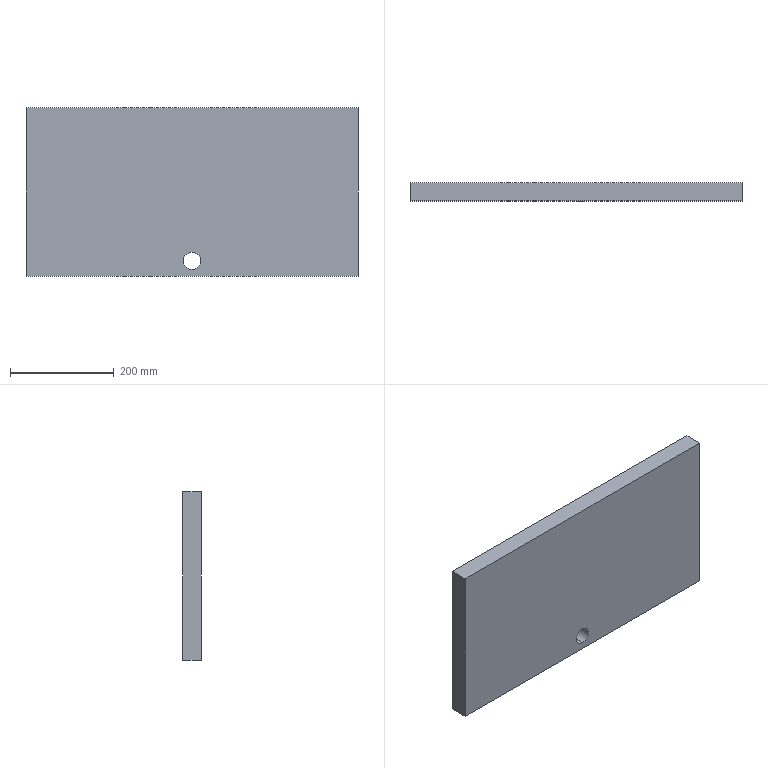Component | SolidWorks | JF21-80.1-1-3(_)-1-SOLID49-1 | 1 solid | 8 faces | box 640 x 35 x 325 mm | volume 7250065 mm3 | plane 6 | cylinder 2 | commonest cylinder face diameters 33 x2
STEP:
#1=COLOUR_RGB('',0.7922,0.8196,0.9333);
#2=FILL_AREA_STYLE_COLOUR('',#1);
#3=FILL_AREA_STYLE('',(#2));
#4=SURFACE_STYLE_FILL_AREA(#3);
#5=SURFACE_SIDE_STYLE('',(#4));
#6=SURFACE_STYLE_USAGE(.BOTH.,#5);
#7=PRESENTATION_STYLE_ASSIGNMENT((#6));
#8=CARTESIAN_POINT('',(0.,-64.567,9.39));
#9=VERTEX_POINT('',#8);
#10=CARTESIAN_POINT('',(0.,-64.567,10.689));
#11=VERTEX_POINT('',#10);
#12=CARTESIAN_POINT('',(0.,-64.567,10.039));
#13=DIRECTION('',(0.,1.,0.));
#14=DIRECTION('',(0.,0.,1.));
#15=AXIS2_PLACEMENT_3D('',#12,#13,#14);
#16=CIRCLE('',#15,0.6496);
#17=EDGE_CURVE('',#9,#11,#16,.T.);
#18=ORIENTED_EDGE('',*,*,#17,.F.);
#19=CARTESIAN_POINT('',(0.,-63.189,9.39));
#20=VERTEX_POINT('',#19);
#21=CARTESIAN_POINT('',(0.,-62.205,9.39));
#22=DIRECTION('',(0.,1.,0.));
#23=VECTOR('',#22,39.37);
#24=LINE('',#21,#23);
#25=EDGE_CURVE('',#9,#20,#24,.T.);
#26=ORIENTED_EDGE('',*,*,#25,.T.);
#27=CARTESIAN_POINT('',(0.,-63.189,10.689));
#28=VERTEX_POINT('',#27);
#29=CARTESIAN_POINT('',(0.,-63.189,10.039));
#30=DIRECTION('',(0.,1.,0.));
#31=DIRECTION('',(0.,0.,1.));
#32=AXIS2_PLACEMENT_3D('',#29,#30,#31);
#33=CIRCLE('',#32,0.6496);
#34=EDGE_CURVE('',#20,#28,#33,.T.);
#35=ORIENTED_EDGE('',*,*,#34,.T.);
#36=CARTESIAN_POINT('',(0.,-62.205,10.689));
#37=DIRECTION('',(0.,1.,0.));
#38=VECTOR('',#37,39.37);
#39=LINE('',#36,#38);
#40=EDGE_CURVE('',#11,#28,#39,.T.);
#41=ORIENTED_EDGE('',*,*,#40,.F.);
#42=EDGE_LOOP('',(#18,#26,#35,#41));
#43=FACE_OUTER_BOUND('',#42,.T.);
#44=CARTESIAN_POINT('',(0.,-62.205,10.039));
#45=DIRECTION('',(0.,1.,0.));
#46=DIRECTION('',(0.,0.,-1.));
#47=AXIS2_PLACEMENT_3D('',#44,#45,#46);
#48=CYLINDRICAL_SURFACE('',#47,0.6496);
#49=ADVANCED_FACE('',(#43),#48,.F.);
#50=CARTESIAN_POINT('',(-12.598,-63.189,8.858));
#51=VERTEX_POINT('',#50);
#52=CARTESIAN_POINT('',(-12.598,-63.189,21.654));
#53=VERTEX_POINT('',#52);
#54=CARTESIAN_POINT('',(-12.598,-63.189,8.858));
#55=DIRECTION('',(0.,0.,1.));
#56=VECTOR('',#55,39.37);
#57=LINE('',#54,#56);
#58=EDGE_CURVE('',#51,#53,#57,.T.);
#59=ORIENTED_EDGE('',*,*,#58,.F.);
#60=CARTESIAN_POINT('',(-12.598,-64.567,8.858));
#61=VERTEX_POINT('',#60);
#62=CARTESIAN_POINT('',(-12.598,-64.567,8.858));
#63=DIRECTION('',(0.,1.,0.));
#64=VECTOR('',#63,39.37);
#65=LINE('',#62,#64);
#66=EDGE_CURVE('',#61,#51,#65,.T.);
#67=ORIENTED_EDGE('',*,*,#66,.F.);
#68=CARTESIAN_POINT('',(-12.598,-64.567,21.654));
#69=VERTEX_POINT('',#68);
#70=CARTESIAN_POINT('',(-12.598,-64.567,8.858));
#71=DIRECTION('',(0.,0.,1.));
#72=VECTOR('',#71,39.37);
#73=LINE('',#70,#72);
#74=EDGE_CURVE('',#61,#69,#73,.T.);
#75=ORIENTED_EDGE('',*,*,#74,.T.);
#76=CARTESIAN_POINT('',(-12.598,-64.567,21.654));
#77=DIRECTION('',(0.,1.,0.));
#78=VECTOR('',#77,39.37);
#79=LINE('',#76,#78);
#80=EDGE_CURVE('',#69,#53,#79,.T.);
#81=ORIENTED_EDGE('',*,*,#80,.T.);
#82=EDGE_LOOP('',(#59,#67,#75,#81));
#83=FACE_OUTER_BOUND('',#82,.T.);
#84=CARTESIAN_POINT('',(-12.598,-64.567,8.858));
#85=DIRECTION('',(-1.,0.,0.));
#86=DIRECTION('',(0.,0.,-1.));
#87=AXIS2_PLACEMENT_3D('',#84,#85,#86);
#88=PLANE('',#87);
#89=ADVANCED_FACE('',(#83),#88,.T.);
#90=CARTESIAN_POINT('',(12.598,-63.189,8.858));
#91=VERTEX_POINT('',#90);
#92=CARTESIAN_POINT('',(-12.598,-63.189,8.858));
#93=DIRECTION('',(-1.,0.,0.));
#94=VECTOR('',#93,39.37);
#95=LINE('',#92,#94);
#96=EDGE_CURVE('',#91,#51,#95,.T.);
#97=ORIENTED_EDGE('',*,*,#96,.F.);
#98=CARTESIAN_POINT('',(12.598,-64.567,8.858));
#99=VERTEX_POINT('',#98);
#100=CARTESIAN_POINT('',(12.598,-64.567,8.858));
#101=DIRECTION('',(0.,1.,0.));
#102=VECTOR('',#101,39.37);
#103=LINE('',#100,#102);
#104=EDGE_CURVE('',#99,#91,#103,.T.);
#105=ORIENTED_EDGE('',*,*,#104,.F.);
#106=CARTESIAN_POINT('',(-12.598,-64.567,8.858));
#107=DIRECTION('',(-1.,0.,0.));
#108=VECTOR('',#107,39.37);
#109=LINE('',#106,#108);
#110=EDGE_CURVE('',#99,#61,#109,.T.);
#111=ORIENTED_EDGE('',*,*,#110,.T.);
#112=ORIENTED_EDGE('',*,*,#66,.T.);
#113=EDGE_LOOP('',(#97,#105,#111,#112));
#114=FACE_OUTER_BOUND('',#113,.T.);
#115=CARTESIAN_POINT('',(-12.598,-64.567,8.858));
#116=DIRECTION('',(-0.,0.,-1.));
#117=DIRECTION('',(1.,0.,-0.));
#118=AXIS2_PLACEMENT_3D('',#115,#116,#117);
#119=PLANE('',#118);
#120=ADVANCED_FACE('',(#114),#119,.T.);
#121=CARTESIAN_POINT('',(12.598,-63.189,21.654));
#122=VERTEX_POINT('',#121);
#123=CARTESIAN_POINT('',(12.598,-63.189,8.858));
#124=DIRECTION('',(0.,0.,-1.));
#125=VECTOR('',#124,39.37);
#126=LINE('',#123,#125);
#127=EDGE_CURVE('',#122,#91,#126,.T.);
#128=ORIENTED_EDGE('',*,*,#127,.F.);
#129=CARTESIAN_POINT('',(12.598,-64.567,21.654));
#130=VERTEX_POINT('',#129);
#131=CARTESIAN_POINT('',(12.598,-64.567,21.654));
#132=DIRECTION('',(0.,1.,0.));
#133=VECTOR('',#132,39.37);
#134=LINE('',#131,#133);
#135=EDGE_CURVE('',#130,#122,#134,.T.);
#136=ORIENTED_EDGE('',*,*,#135,.F.);
#137=CARTESIAN_POINT('',(12.598,-64.567,8.858));
#138=DIRECTION('',(0.,0.,-1.));
#139=VECTOR('',#138,39.37);
#140=LINE('',#137,#139);
#141=EDGE_CURVE('',#130,#99,#140,.T.);
#142=ORIENTED_EDGE('',*,*,#141,.T.);
#143=ORIENTED_EDGE('',*,*,#104,.T.);
#144=EDGE_LOOP('',(#128,#136,#142,#143));
#145=FACE_OUTER_BOUND('',#144,.T.);
#146=CARTESIAN_POINT('',(12.598,-64.567,8.858));
#147=DIRECTION('',(1.,0.,0.));
#148=DIRECTION('',(0.,0.,1.));
#149=AXIS2_PLACEMENT_3D('',#146,#147,#148);
#150=PLANE('',#149);
#151=ADVANCED_FACE('',(#145),#150,.T.);
#152=CARTESIAN_POINT('',(-12.598,-63.189,21.654));
#153=DIRECTION('',(1.,0.,0.));
#154=VECTOR('',#153,39.37);
#155=LINE('',#152,#154);
#156=EDGE_CURVE('',#53,#122,#155,.T.);
#157=ORIENTED_EDGE('',*,*,#156,.F.);
#158=ORIENTED_EDGE('',*,*,#80,.F.);
#159=CARTESIAN_POINT('',(-12.598,-64.567,21.654));
#160=DIRECTION('',(1.,0.,0.));
#161=VECTOR('',#160,39.37);
#162=LINE('',#159,#161);
#163=EDGE_CURVE('',#69,#130,#162,.T.);
#164=ORIENTED_EDGE('',*,*,#163,.T.);
#165=ORIENTED_EDGE('',*,*,#135,.T.);
#166=EDGE_LOOP('',(#157,#158,#164,#165));
#167=FACE_OUTER_BOUND('',#166,.T.);
#168=CARTESIAN_POINT('',(-12.598,-64.567,21.654));
#169=DIRECTION('',(0.,0.,1.));
#170=DIRECTION('',(-1.,0.,0.));
#171=AXIS2_PLACEMENT_3D('',#168,#169,#170);
#172=PLANE('',#171);
#173=ADVANCED_FACE('',(#167),#172,.T.);
#174=CARTESIAN_POINT('',(0.,-64.567,10.039));
#175=DIRECTION('',(0.,1.,0.));
#176=DIRECTION('',(0.,0.,1.));
#177=AXIS2_PLACEMENT_3D('',#174,#175,#176);
#178=CIRCLE('',#177,0.6496);
#179=EDGE_CURVE('',#11,#9,#178,.T.);
#180=ORIENTED_EDGE('',*,*,#179,.T.);
#181=ORIENTED_EDGE('',*,*,#17,.T.);
#182=EDGE_LOOP('',(#180,#181));
#183=FACE_BOUND('',#182,.T.);
#184=ORIENTED_EDGE('',*,*,#74,.F.);
#185=ORIENTED_EDGE('',*,*,#110,.F.);
#186=ORIENTED_EDGE('',*,*,#141,.F.);
#187=ORIENTED_EDGE('',*,*,#163,.F.);
#188=EDGE_LOOP('',(#184,#185,#186,#187));
#189=FACE_OUTER_BOUND('',#188,.T.);
#190=CARTESIAN_POINT('',(-12.598,-64.567,21.654));
#191=DIRECTION('',(0.,1.,0.));
#192=DIRECTION('',(0.,0.,-1.));
#193=AXIS2_PLACEMENT_3D('',#190,#191,#192);
#194=PLANE('',#193);
#195=ADVANCED_FACE('',(#183,#189),#194,.F.);
#196=CARTESIAN_POINT('',(0.,-63.189,10.039));
#197=DIRECTION('',(0.,1.,0.));
#198=DIRECTION('',(0.,0.,1.));
#199=AXIS2_PLACEMENT_3D('',#196,#197,#198);
#200=CIRCLE('',#199,0.6496);
#201=EDGE_CURVE('',#28,#20,#200,.T.);
#202=ORIENTED_EDGE('',*,*,#201,.F.);
#203=ORIENTED_EDGE('',*,*,#34,.F.);
#204=EDGE_LOOP('',(#202,#203));
#205=FACE_BOUND('',#204,.T.);
#206=ORIENTED_EDGE('',*,*,#58,.T.);
#207=ORIENTED_EDGE('',*,*,#156,.T.);
#208=ORIENTED_EDGE('',*,*,#127,.T.);
#209=ORIENTED_EDGE('',*,*,#96,.T.);
#210=EDGE_LOOP('',(#206,#207,#208,#209));
#211=FACE_OUTER_BOUND('',#210,.T.);
#212=CARTESIAN_POINT('',(-12.598,-63.189,21.654));
#213=DIRECTION('',(0.,1.,0.));
#214=DIRECTION('',(0.,0.,-1.));
#215=AXIS2_PLACEMENT_3D('',#212,#213,#214);
#216=PLANE('',#215);
#217=ADVANCED_FACE('',(#205,#211),#216,.T.);
#218=ORIENTED_EDGE('',*,*,#25,.F.);
#219=ORIENTED_EDGE('',*,*,#179,.F.);
#220=ORIENTED_EDGE('',*,*,#40,.T.);
#221=ORIENTED_EDGE('',*,*,#201,.T.);
#222=EDGE_LOOP('',(#218,#219,#220,#221));
#223=FACE_OUTER_BOUND('',#222,.T.);
#224=CARTESIAN_POINT('',(0.,-62.205,10.039));
#225=DIRECTION('',(0.,1.,0.));
#226=DIRECTION('',(0.,0.,-1.));
#227=AXIS2_PLACEMENT_3D('',#224,#225,#226);
#228=CYLINDRICAL_SURFACE('',#227,0.6496);
#229=ADVANCED_FACE('',(#223),#228,.F.);
#230=CLOSED_SHELL('',(#49,#89,#120,#151,#173,#195,#217,#229));
#231=MANIFOLD_SOLID_BREP('',#230);
#232=STYLED_ITEM('',(#7),#231);
#233=(LENGTH_UNIT()NAMED_UNIT(*)SI_UNIT($,.METRE.));
#234=LENGTH_MEASURE_WITH_UNIT(LENGTH_MEASURE(0.0254),#233);
#235=DIMENSIONAL_EXPONENTS(1.,0.,0.,0.,0.,0.,0.);
#236=(CONVERSION_BASED_UNIT('',#234)LENGTH_UNIT()NAMED_UNIT(#235));
#237=UNCERTAINTY_MEASURE_WITH_UNIT(LENGTH_MEASURE(0.00001),#236,'','');
#238=(NAMED_UNIT(*)PLANE_ANGLE_UNIT()SI_UNIT($,.RADIAN.));
#239=(NAMED_UNIT(*)SI_UNIT($,.STERADIAN.)SOLID_ANGLE_UNIT());
#240=(GEOMETRIC_REPRESENTATION_CONTEXT(3)GLOBAL_UNCERTAINTY_ASSIGNED_CONTEXT((#237))GLOBAL_UNIT_ASSIGNED_CONTEXT((#236,#238,#239))REPRESENTATION_CONTEXT('',''));
#241=MECHANICAL_DESIGN_GEOMETRIC_PRESENTATION_REPRESENTATION('',(#232),#240);
#242=CARTESIAN_POINT('',(0.,0.,0.));
#243=DIRECTION('',(0.,0.,1.));
#244=DIRECTION('',(1.,0.,0.));
#245=AXIS2_PLACEMENT_3D('',#242,#243,#244);
#246=(LENGTH_UNIT()NAMED_UNIT(*)SI_UNIT($,.METRE.));
#247=LENGTH_MEASURE_WITH_UNIT(LENGTH_MEASURE(0.0254),#246);
#248=DIMENSIONAL_EXPONENTS(1.,0.,0.,0.,0.,0.,0.);
#249=(CONVERSION_BASED_UNIT('',#247)LENGTH_UNIT()NAMED_UNIT(#248));
#250=UNCERTAINTY_MEASURE_WITH_UNIT(LENGTH_MEASURE(0.00001),#249,'','');
#251=(NAMED_UNIT(*)PLANE_ANGLE_UNIT()SI_UNIT($,.RADIAN.));
#252=(NAMED_UNIT(*)SI_UNIT($,.STERADIAN.)SOLID_ANGLE_UNIT());
#253=(GEOMETRIC_REPRESENTATION_CONTEXT(3)GLOBAL_UNCERTAINTY_ASSIGNED_CONTEXT((#250))GLOBAL_UNIT_ASSIGNED_CONTEXT((#249,#251,#252))REPRESENTATION_CONTEXT('',''));
#254=ADVANCED_BREP_SHAPE_REPRESENTATION('',(#231,#245),#253);
#255=PRESENTATION_LAYER_ASSIGNMENT('','',(#232));